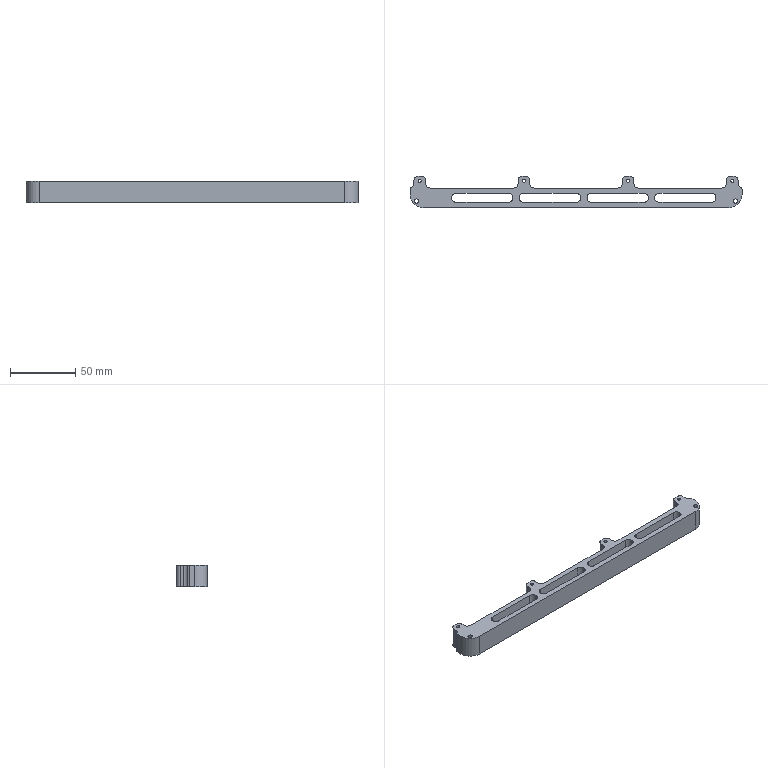CAM job | Mastercam | mm | 10 operations | part box 255 x 24 x 16.7
1. Facing | 24 - 100 平铣刀
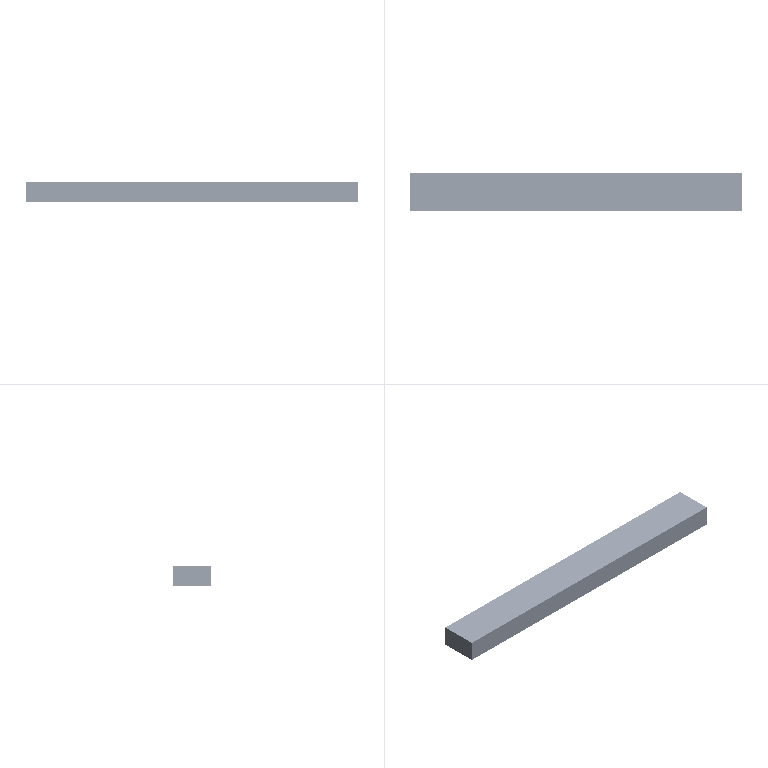2. 2D High Speed (2D Dynamic Mill) | 10 - 10 平铣刀
3. Contour (Remachining) | 6 - 6 平铣刀
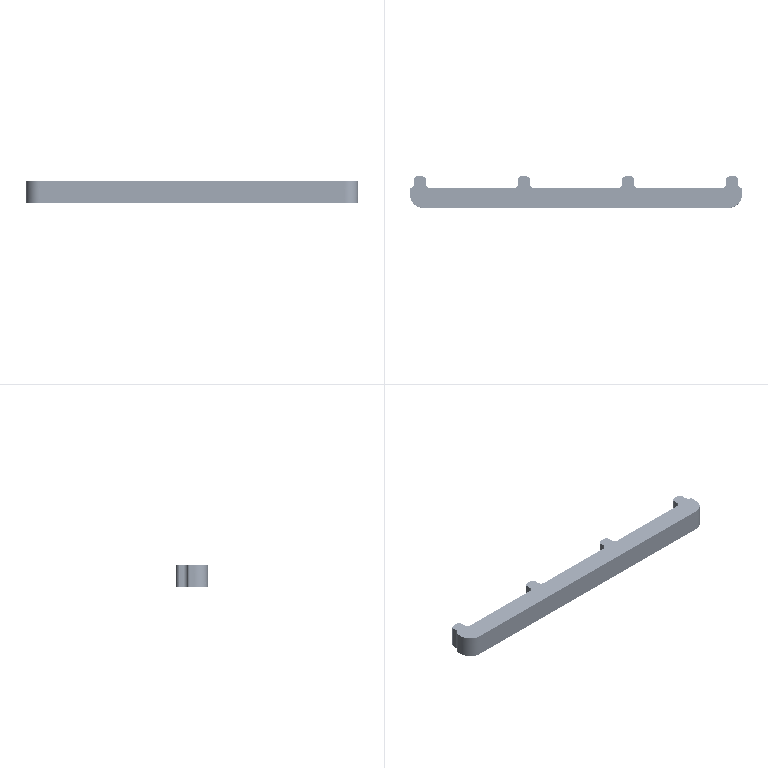4. Contour (Ramp) | 6 - 6 平铣刀
5. Contour (2D) | 6 - 6 平铣刀
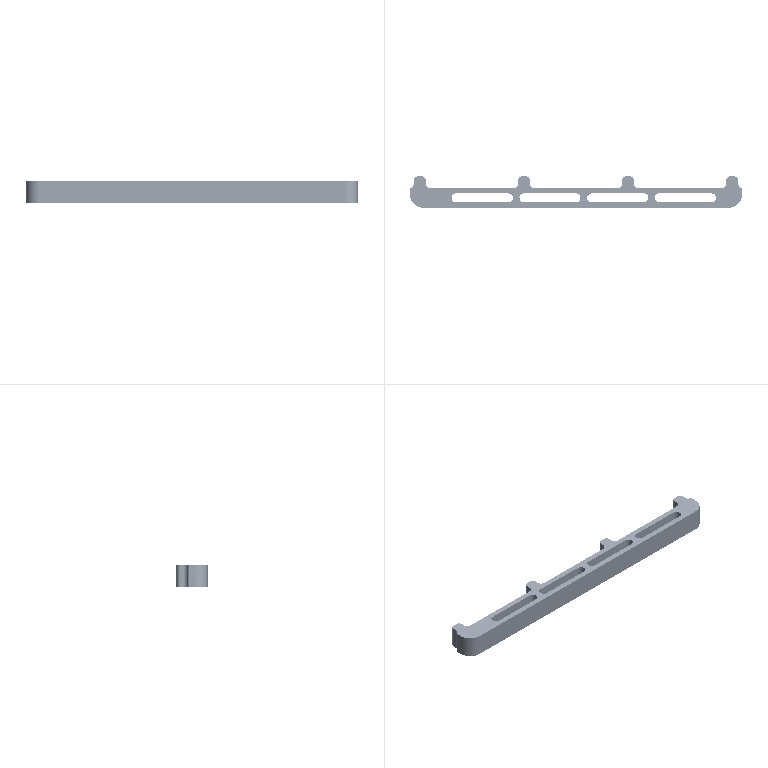6. Contour (Ramp) | 6 - 6 平铣刀
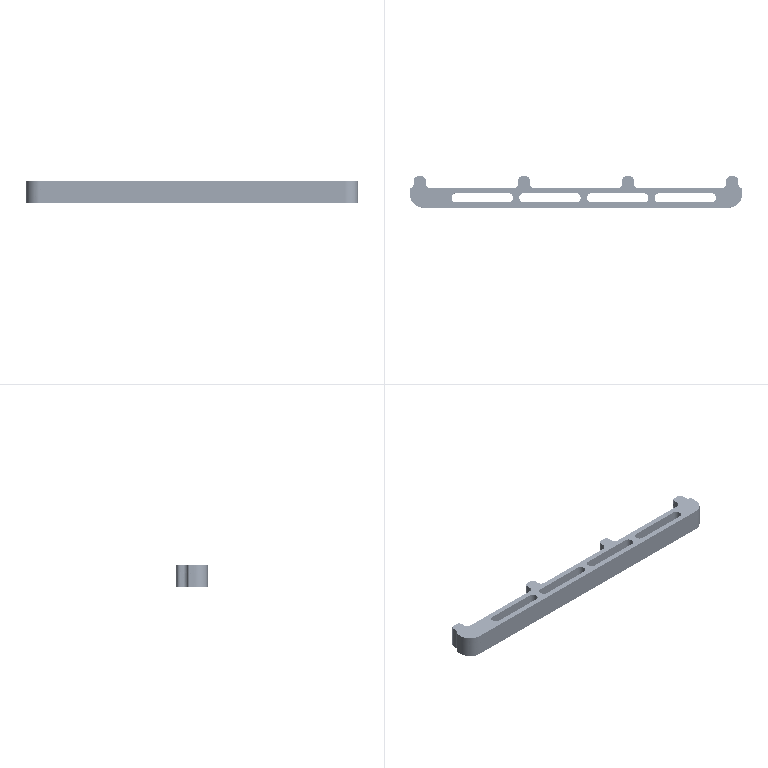7. Drill/Counterbore | 7 - 4 倒角刀
8. Contour (2D chamfer) | 7 - 4 倒角刀
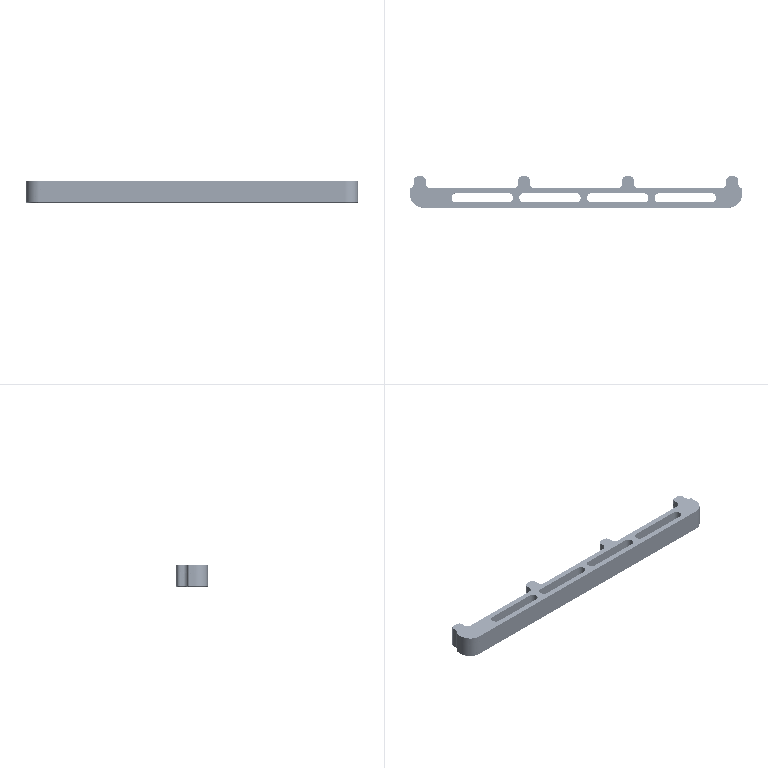9. Facing | 24 - 100 平铣刀
10. Contour (2D chamfer) | 7 - 4 倒角刀